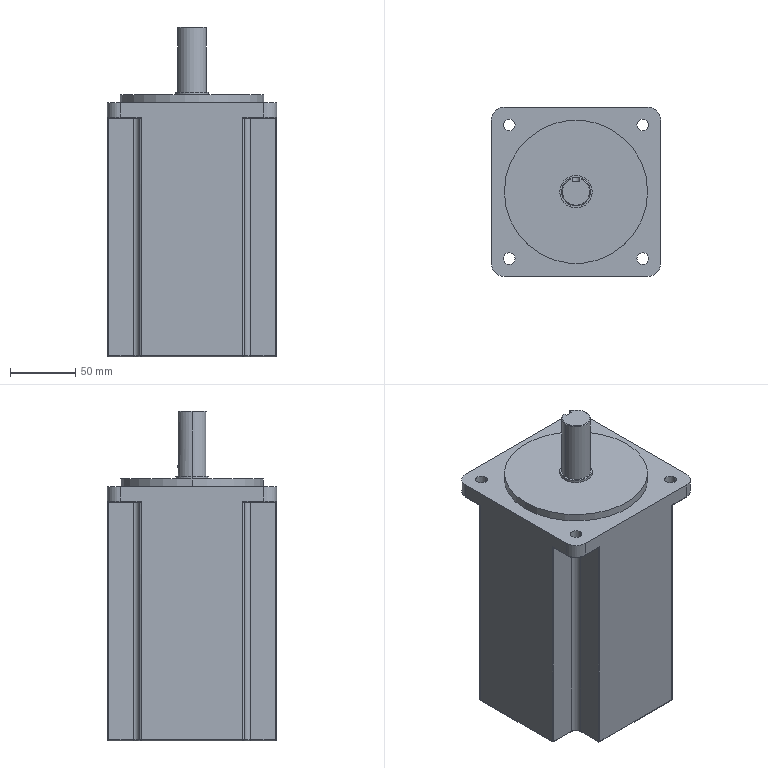Component | SolidWorks | ServoMotor130SJT-M075D(AZ)-1 | 1 solid | 102 faces | volume 2908860 mm3 | cylinder 55 | plane 26 | torus 10 | sphere 8 | cone 3 | commonest cylinder face diameters 2 x28 9 x8 20 x6 10 x4 30 x2 25 x2 110 x2 22 x2 | material Plain Carbon Steel